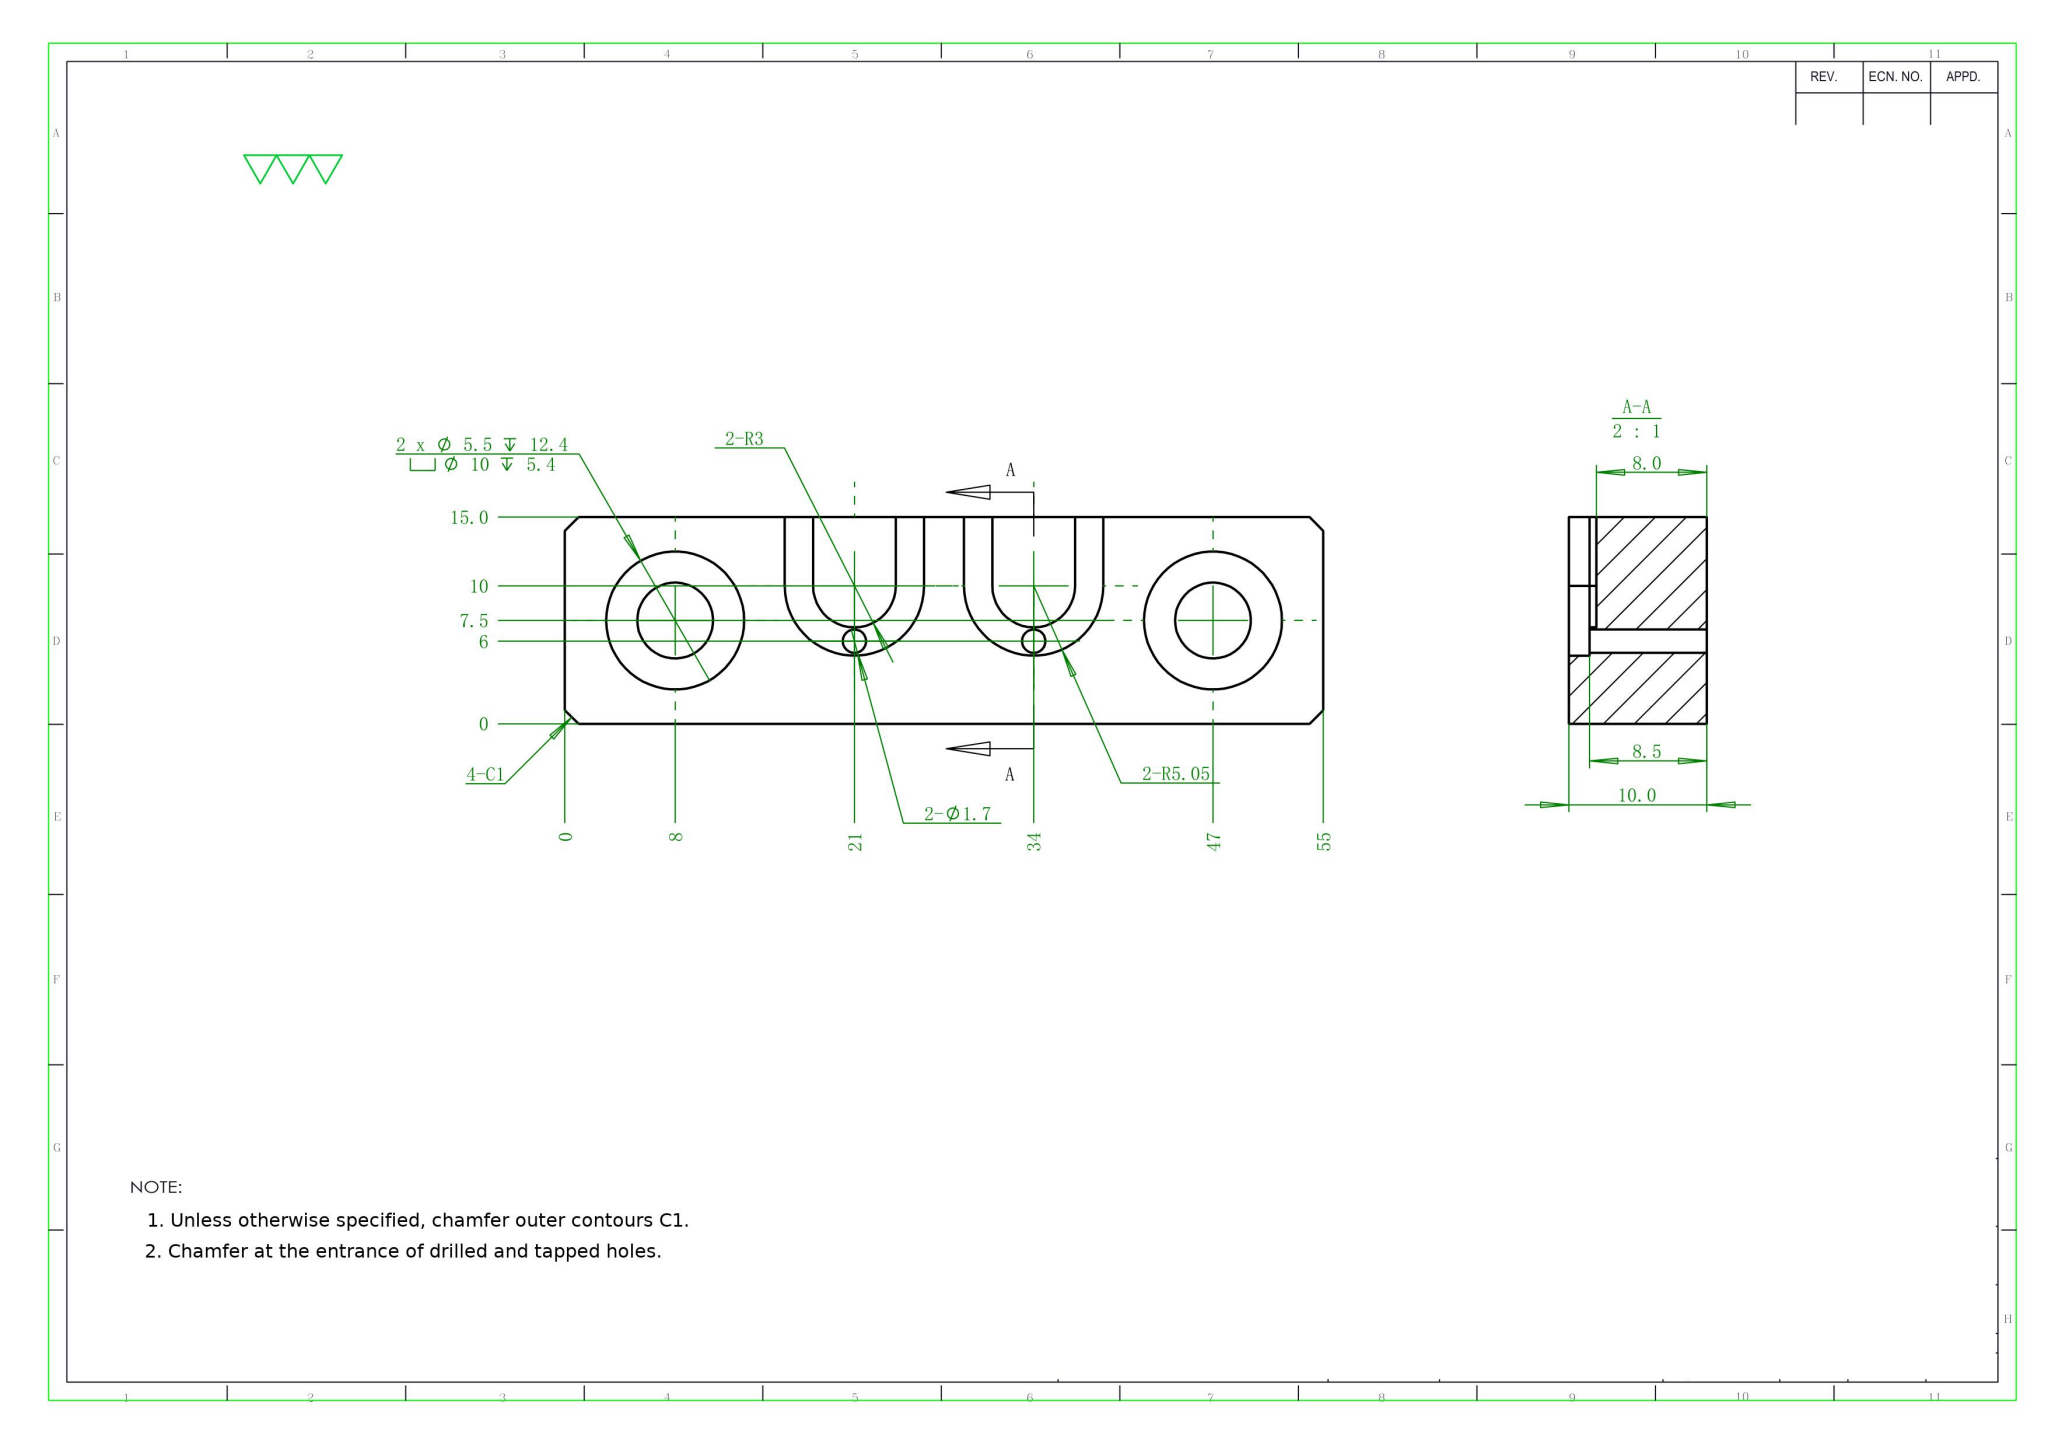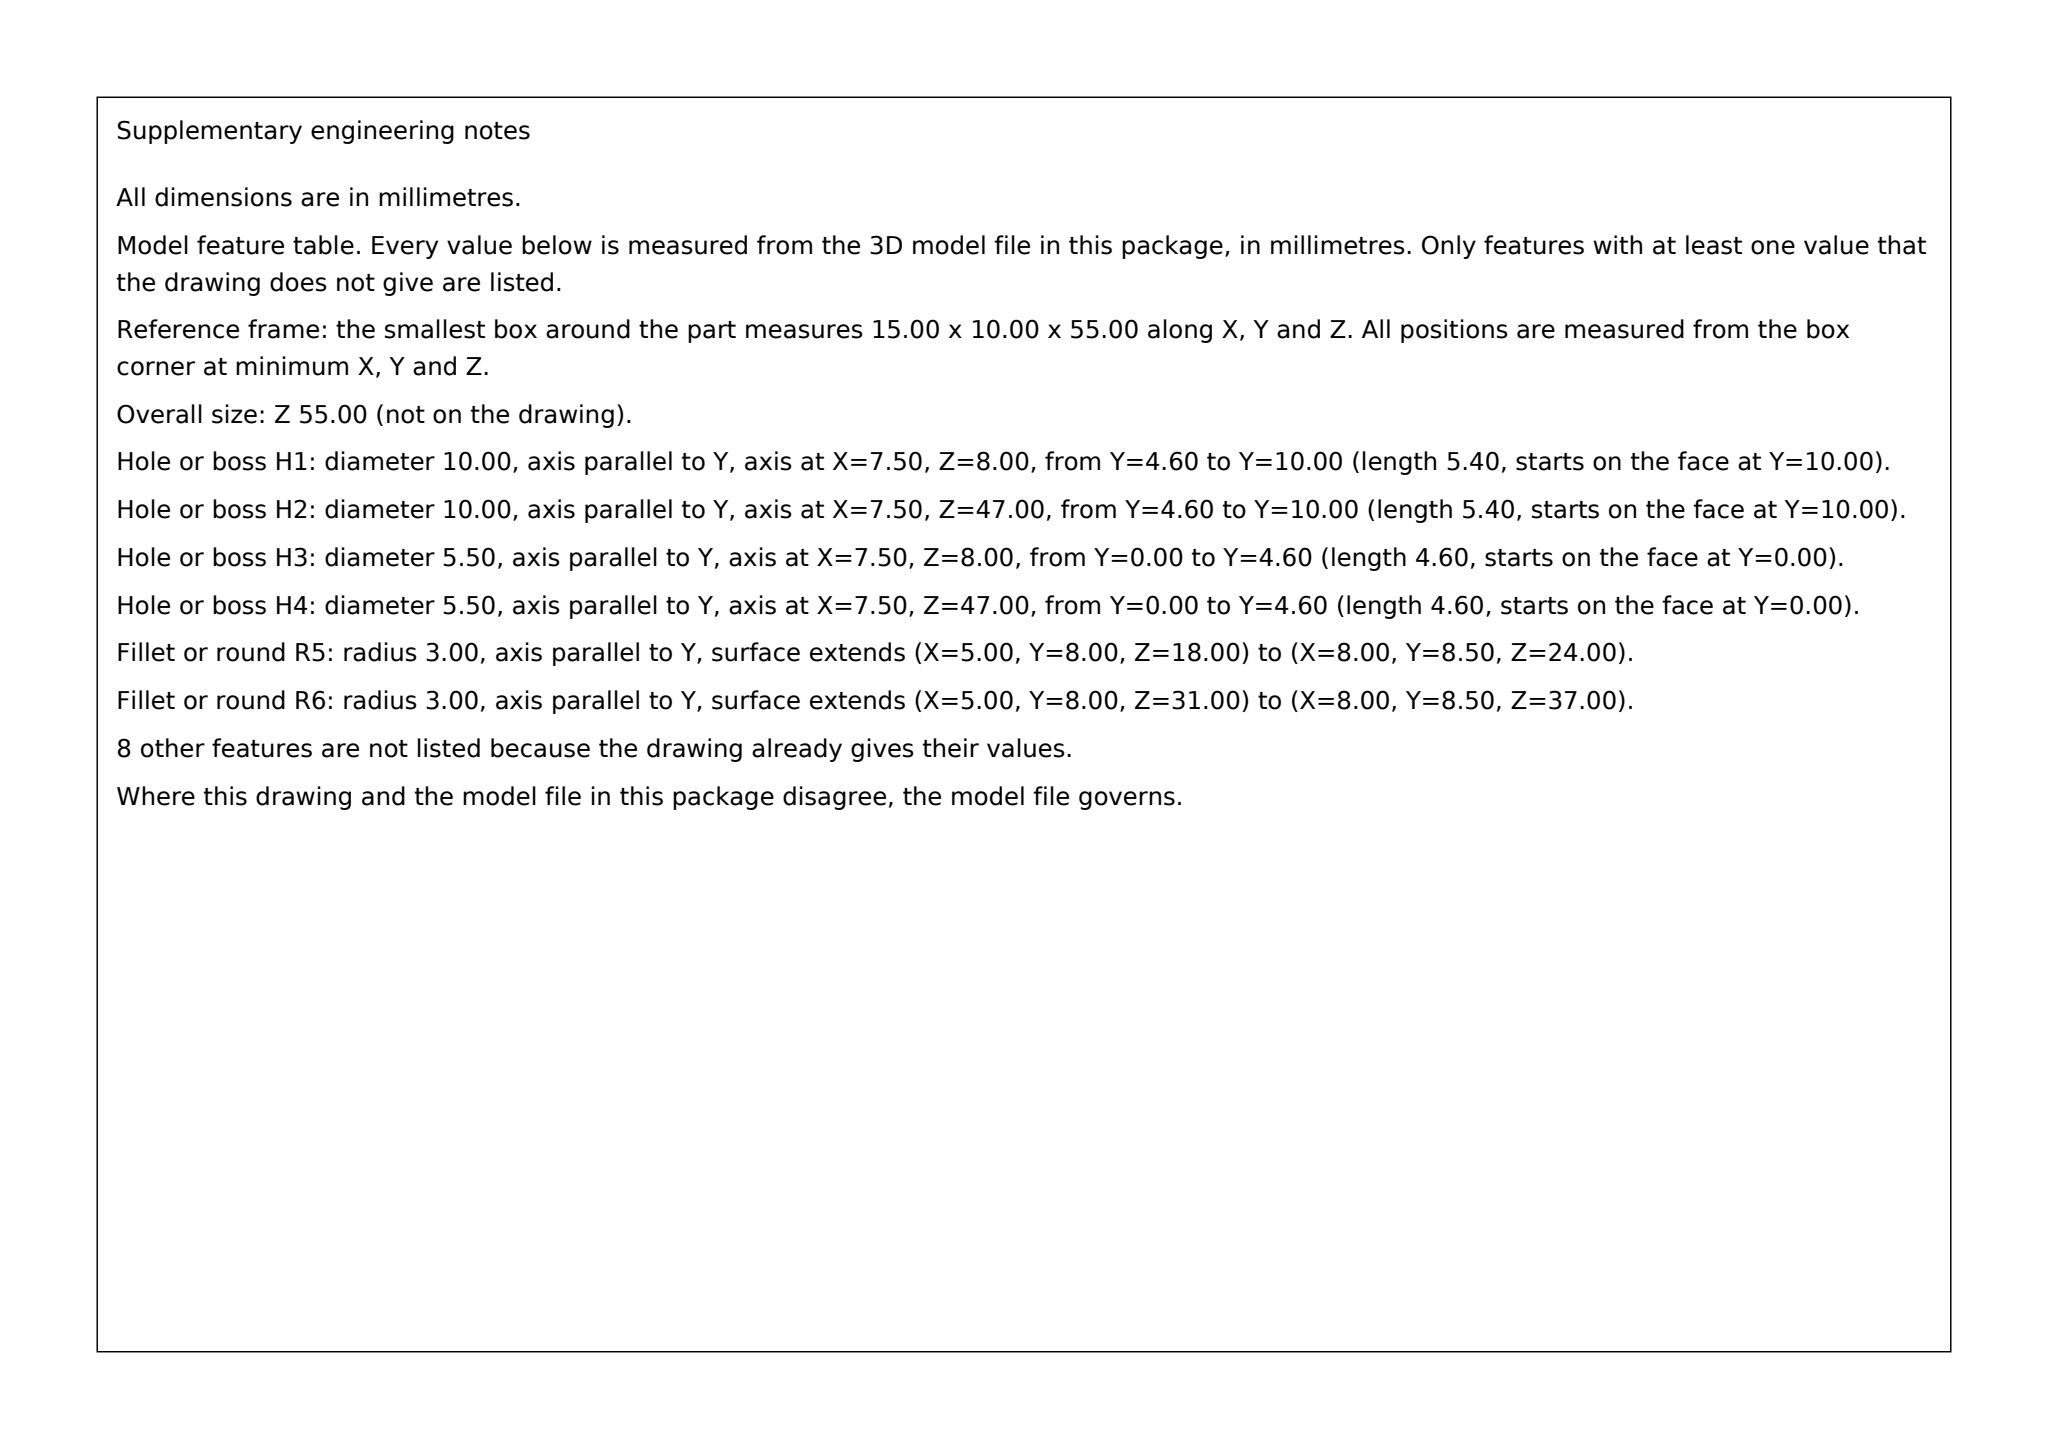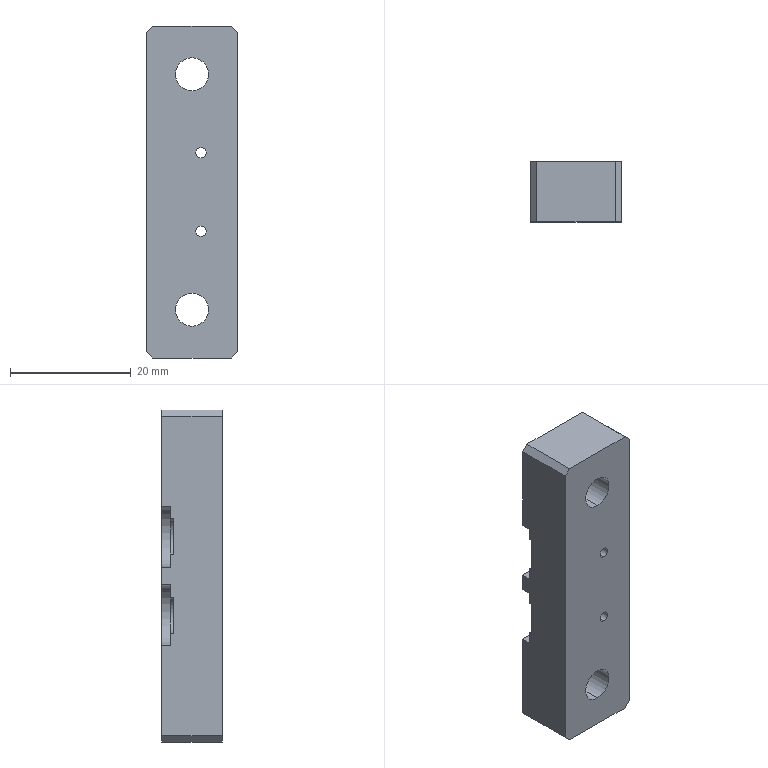Part | SolidWorks | mm | 1 solid | 40 faces | box 15 x 10 x 55 mm | volume 6809 mm3 | plane 24 | cylinder 16 | commonest cylinder face diameters 1.7 x4 10 x4 5.5 x4 10.1 x2 6 x2
build123d program:
from build123d import *

# Parameters (mm, degrees)
SKETCH1_W                                       = 15
SKETCH1_H                                       = 55
BOSS_EXTRUDE1_DEPTH                             = 10
CUT_EXTRUDE1_DEPTH                              = 1.5
CUT_EXTRUDE2_DEPTH                              = 0.5
M5_HEX_SOCKET_HEAD_CAP_SCREW_CBORE1_D           = 5.5
M5_HEX_SOCKET_HEAD_CAP_SCREW_CBORE1_DEPTH       = 12.4
M5_HEX_SOCKET_HEAD_CAP_SCREW_CBORE1_CBORE_D     = 10
M5_HEX_SOCKET_HEAD_CAP_SCREW_CBORE1_CBORE_DEPTH = 5.4
M5_HEX_SOCKET_HEAD_CAP_SCREW_CBORE1_TIP         = 1.652
SKETCH12_R                                      = 0.85
CUT_EXTRUDE10_DEPTH                             = 31.208
CHAMFER1_SIZE                                   = 1


with BuildPart() as part:
    # Sketch1 → Boss-Extrude1 (new body)
    with BuildSketch(Plane(origin=(0, 0, 0), x_dir=(1, 0, 0), z_dir=(0, 1, 0))):
        Rectangle(SKETCH1_W, SKETCH1_H)
    extrude(amount=BOSS_EXTRUDE1_DEPTH)

    # Sketch7 → Cut-Extrude1 (cut)
    with BuildSketch(Plane(origin=(0, 10, 0), x_dir=(1, 0, 0), z_dir=(0, 1, 0))):
        with BuildLine():
            Line((-7.5, 11.55), (-2.5, 11.55))
            ThreePointArc((-2.5, 11.55), (2.55, 6.5), (-2.5, 1.45))
            Line((-2.5, 1.45), (-7.5, 1.45))
            ThreePointArc((-7.5, 1.45), (-12.55, 6.5), (-7.5, 11.55))
        make_face()
        with BuildLine():
            Line((-7.5, -11.55), (-2.5, -11.55))
            ThreePointArc((-2.5, -11.55), (2.55, -6.5), (-2.5, -1.45))
            Line((-2.5, -1.45), (-7.5, -1.45))
            ThreePointArc((-7.5, -1.45), (-12.55, -6.5), (-7.5, -11.55))
        make_face()
    extrude(amount=-CUT_EXTRUDE1_DEPTH, mode=Mode.SUBTRACT)

    # Sketch9 → Cut-Extrude2 (cut)
    with BuildSketch(Plane(origin=(0, 8.5, 0), x_dir=(1, 0, 0), z_dir=(0, 1, 0))):
        with BuildLine():
            Line((-2.5, 3.5), (-7.5, 3.5))
            ThreePointArc((-7.5, 3.5), (-10.5, 6.5), (-7.5, 9.5))
            Line((-7.5, 9.5), (-2.5, 9.5))
            ThreePointArc((-2.5, 9.5), (0.5, 6.5), (-2.5, 3.5))
        make_face()
        with BuildLine():
            Line((-2.5, -3.5), (-7.5, -3.5))
            ThreePointArc((-7.5, -3.5), (-10.5, -6.5), (-7.5, -9.5))
            Line((-7.5, -9.5), (-2.5, -9.5))
            ThreePointArc((-2.5, -9.5), (0.5, -6.5), (-2.5, -3.5))
        make_face()
    extrude(amount=-CUT_EXTRUDE2_DEPTH, mode=Mode.SUBTRACT)

    # M5 Hex Socket Head Cap Screw CBORE1
    with Locations(Plane(origin=(0, 10, 0), x_dir=(1, 0, 0), z_dir=(0, 1, 0))):
        with Locations((0, 19.5), (0, -19.5)):
            CounterBoreHole(M5_HEX_SOCKET_HEAD_CAP_SCREW_CBORE1_D / 2, M5_HEX_SOCKET_HEAD_CAP_SCREW_CBORE1_CBORE_D / 2, M5_HEX_SOCKET_HEAD_CAP_SCREW_CBORE1_CBORE_DEPTH, depth=M5_HEX_SOCKET_HEAD_CAP_SCREW_CBORE1_DEPTH)
            with Locations((0, 0, -(M5_HEX_SOCKET_HEAD_CAP_SCREW_CBORE1_DEPTH + M5_HEX_SOCKET_HEAD_CAP_SCREW_CBORE1_TIP / 2))):  # 118° drill point
                Cone(0, M5_HEX_SOCKET_HEAD_CAP_SCREW_CBORE1_D / 2, M5_HEX_SOCKET_HEAD_CAP_SCREW_CBORE1_TIP, mode=Mode.SUBTRACT)

    # Sketch12 → Cut-Extrude10 (cut, through all)
    with BuildSketch(Plane(origin=(0, 0, 0), x_dir=(1, 0, 0), z_dir=(0, 1, 0))):
        with Locations(Location((1.5, -6.5, 0), (0, 0, 90))):
            Circle(SKETCH12_R)
        with Locations(Location((1.5, 6.5, 0), (0, 0, 90))):
            Circle(SKETCH12_R)
    extrude(amount=CUT_EXTRUDE10_DEPTH, mode=Mode.SUBTRACT)

    # Chamfer1
    chamfer1_edges = [part.edges().sort_by_distance(p)[0] for p in [
        (7.5, 5, 27.5),
        (-7.5, 5, 27.5),
        (-7.5, 5, -27.5),
        (7.5, 5, -27.5),
    ]]
    chamfer(chamfer1_edges, length=CHAMFER1_SIZE)


solid = part.part